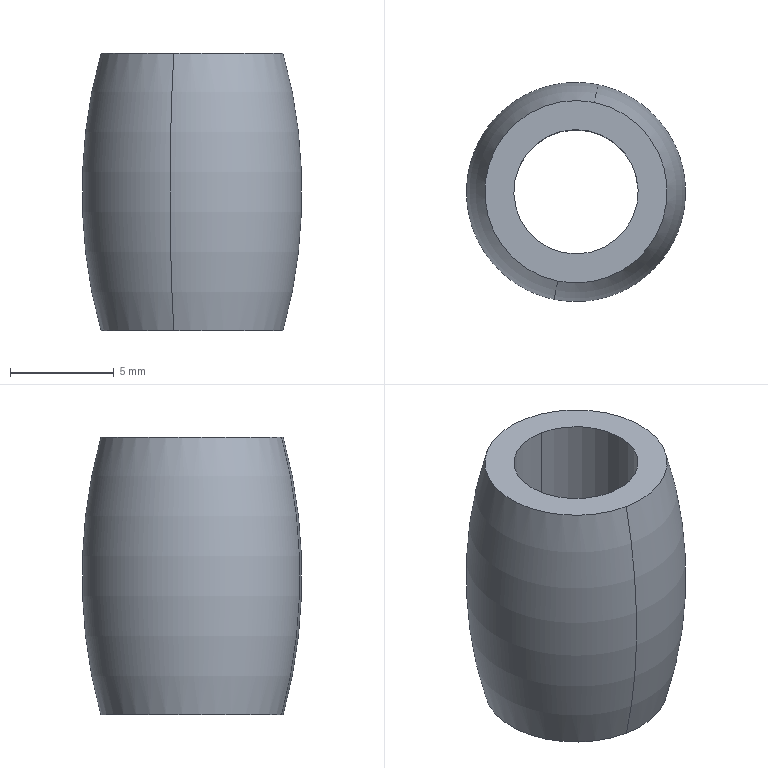Component | SolidWorks | Half-1_Roller-2 | 1 solid | 6 faces | volume 678 mm3 | cylinder 2 | plane 2 | torus 2 | commonest cylinder face diameters 6 x2 | material Rubber
build123d program:
from build123d import *

# Parameters (mm, degrees)
SKETCH2_R          = 3
CUT_EXTRUDE3_DEPTH = 30.203


with BuildPart() as part:
    # Sketch1 → Revolve1 (revolve)
    with BuildSketch(Plane.XY):
        with BuildLine():
            Line((-47.251, 20.1), (-33.851, 20.1))
            Line((-33.851, 20.1), (-33.851, 24.5))
            ThreePointArc((-33.851, 24.5), (-40.551, 25.4), (-47.251, 24.5))
            Line((-47.251, 24.5), (-47.251, 20.1))
        make_face()
    revolve(axis=Axis((-1.751, 20.1, 0), (-1, 0, 0)))

    # Sketch2 → Cut-Extrude3 (cut, through all)
    with BuildSketch(Plane(origin=(-33.851, 0, 0), x_dir=(0, 0, -1), z_dir=(1, 0, 0))):
        with Locations(Location((0, 20.1, 0), (0, 0, 90))):
            Circle(SKETCH2_R)
    extrude(amount=-CUT_EXTRUDE3_DEPTH, mode=Mode.SUBTRACT)


solid = part.part

# Placed as in the assembly
solid = solid.moved(Location((-19.269, -22.2, -3.551), (0, 90, 0)))
STEP:
#1=CARTESIAN_POINT('',(-0.7822,-0.1984,1.193));
#2=VERTEX_POINT('',#1);
#3=CARTESIAN_POINT('',(-0.735,0.03304,1.193));
#4=VERTEX_POINT('',#3);
#5=CARTESIAN_POINT('',(-0.7586,-0.08269,1.193));
#6=DIRECTION('',(-0.,-0.,1.));
#7=DIRECTION('',(0.1999,0.9798,0.));
#8=AXIS2_PLACEMENT_3D('',#5,#6,#7);
#9=CIRCLE('',#8,0.1181);
#10=EDGE_CURVE('',#2,#4,#9,.T.);
#11=ORIENTED_EDGE('',*,*,#10,.F.);
#12=CARTESIAN_POINT('',(-0.7822,-0.1984,1.72));
#13=VERTEX_POINT('',#12);
#14=CARTESIAN_POINT('',(-0.7822,-0.1984,1.193));
#15=DIRECTION('',(-0.,-0.,1.));
#16=VECTOR('',#15,39.37);
#17=LINE('',#14,#16);
#18=EDGE_CURVE('',#2,#13,#17,.T.);
#19=ORIENTED_EDGE('',*,*,#18,.T.);
#20=CARTESIAN_POINT('',(-0.735,0.03304,1.72));
#21=VERTEX_POINT('',#20);
#22=CARTESIAN_POINT('',(-0.7586,-0.08269,1.72));
#23=DIRECTION('',(-0.,-0.,1.));
#24=DIRECTION('',(0.1999,0.9798,0.));
#25=AXIS2_PLACEMENT_3D('',#22,#23,#24);
#26=CIRCLE('',#25,0.1181);
#27=EDGE_CURVE('',#13,#21,#26,.T.);
#28=ORIENTED_EDGE('',*,*,#27,.T.);
#29=CARTESIAN_POINT('',(-0.735,0.03304,1.193));
#30=DIRECTION('',(-0.,-0.,1.));
#31=VECTOR('',#30,39.37);
#32=LINE('',#29,#31);
#33=EDGE_CURVE('',#4,#21,#32,.T.);
#34=ORIENTED_EDGE('',*,*,#33,.F.);
#35=EDGE_LOOP('',(#11,#19,#28,#34));
#36=FACE_OUTER_BOUND('',#35,.T.);
#37=CARTESIAN_POINT('',(-0.7586,-0.08269,1.193));
#38=DIRECTION('',(-0.,-0.,1.));
#39=DIRECTION('',(0.1999,0.9798,0.));
#40=AXIS2_PLACEMENT_3D('',#37,#38,#39);
#41=CYLINDRICAL_SURFACE('',#40,0.1181);
#42=ADVANCED_FACE('',(#36),#41,.F.);
#43=CARTESIAN_POINT('',(-0.724,0.08706,1.193));
#44=VERTEX_POINT('',#43);
#45=CARTESIAN_POINT('',(-0.7933,-0.2524,1.193));
#46=VERTEX_POINT('',#45);
#47=CARTESIAN_POINT('',(-0.7586,-0.08269,1.193));
#48=DIRECTION('',(-0.,-0.,1.));
#49=DIRECTION('',(0.1999,0.9798,0.));
#50=AXIS2_PLACEMENT_3D('',#47,#48,#49);
#51=CIRCLE('',#50,0.1732);
#52=EDGE_CURVE('',#44,#46,#51,.T.);
#53=ORIENTED_EDGE('',*,*,#52,.T.);
#54=CARTESIAN_POINT('',(-0.7933,-0.2524,1.72));
#55=VERTEX_POINT('',#54);
#56=CARTESIAN_POINT('',(-0.6004,0.6927,1.457));
#57=DIRECTION('',(-0.9798,0.1999,-0.));
#58=DIRECTION('',(-0.1999,-0.9798,0.));
#59=AXIS2_PLACEMENT_3D('',#56,#57,#58);
#60=CIRCLE('',#59,1.);
#61=EDGE_CURVE('',#46,#55,#60,.T.);
#62=ORIENTED_EDGE('',*,*,#61,.T.);
#63=CARTESIAN_POINT('',(-0.724,0.08706,1.72));
#64=VERTEX_POINT('',#63);
#65=CARTESIAN_POINT('',(-0.7586,-0.08269,1.72));
#66=DIRECTION('',(-0.,-0.,1.));
#67=DIRECTION('',(0.1999,0.9798,0.));
#68=AXIS2_PLACEMENT_3D('',#65,#66,#67);
#69=CIRCLE('',#68,0.1732);
#70=EDGE_CURVE('',#64,#55,#69,.T.);
#71=ORIENTED_EDGE('',*,*,#70,.F.);
#72=CARTESIAN_POINT('',(-0.9168,-0.8581,1.457));
#73=DIRECTION('',(0.9798,-0.1999,0.));
#74=DIRECTION('',(0.1999,0.9798,0.));
#75=AXIS2_PLACEMENT_3D('',#72,#73,#74);
#76=CIRCLE('',#75,1.);
#77=EDGE_CURVE('',#44,#64,#76,.T.);
#78=ORIENTED_EDGE('',*,*,#77,.F.);
#79=EDGE_LOOP('',(#53,#62,#71,#78));
#80=FACE_OUTER_BOUND('',#79,.T.);
#81=CARTESIAN_POINT('',(-0.7586,-0.08269,1.457));
#82=DIRECTION('',(-0.,-0.,1.));
#83=DIRECTION('',(0.1999,0.9798,0.));
#84=AXIS2_PLACEMENT_3D('',#81,#82,#83);
#85=TOROIDAL_SURFACE('',#84,-0.7913,1.);
#86=ADVANCED_FACE('',(#80),#85,.T.);
#87=CARTESIAN_POINT('',(-0.7586,-0.08269,1.72));
#88=DIRECTION('',(-0.,-0.,1.));
#89=DIRECTION('',(0.1999,0.9798,0.));
#90=AXIS2_PLACEMENT_3D('',#87,#88,#89);
#91=CIRCLE('',#90,0.1181);
#92=EDGE_CURVE('',#21,#13,#91,.T.);
#93=ORIENTED_EDGE('',*,*,#92,.F.);
#94=ORIENTED_EDGE('',*,*,#27,.F.);
#95=EDGE_LOOP('',(#93,#94));
#96=FACE_BOUND('',#95,.T.);
#97=ORIENTED_EDGE('',*,*,#70,.T.);
#98=CARTESIAN_POINT('',(-0.7586,-0.08269,1.72));
#99=DIRECTION('',(-0.,-0.,1.));
#100=DIRECTION('',(0.1999,0.9798,0.));
#101=AXIS2_PLACEMENT_3D('',#98,#99,#100);
#102=CIRCLE('',#101,0.1732);
#103=EDGE_CURVE('',#55,#64,#102,.T.);
#104=ORIENTED_EDGE('',*,*,#103,.T.);
#105=EDGE_LOOP('',(#97,#104));
#106=FACE_OUTER_BOUND('',#105,.T.);
#107=CARTESIAN_POINT('',(-0.9168,-0.8581,1.72));
#108=DIRECTION('',(-0.,-0.,1.));
#109=DIRECTION('',(0.1999,0.9798,0.));
#110=AXIS2_PLACEMENT_3D('',#107,#108,#109);
#111=PLANE('',#110);
#112=ADVANCED_FACE('',(#96,#106),#111,.T.);
#113=ORIENTED_EDGE('',*,*,#61,.F.);
#114=CARTESIAN_POINT('',(-0.7586,-0.08269,1.193));
#115=DIRECTION('',(-0.,-0.,1.));
#116=DIRECTION('',(0.1999,0.9798,0.));
#117=AXIS2_PLACEMENT_3D('',#114,#115,#116);
#118=CIRCLE('',#117,0.1732);
#119=EDGE_CURVE('',#46,#44,#118,.T.);
#120=ORIENTED_EDGE('',*,*,#119,.T.);
#121=ORIENTED_EDGE('',*,*,#77,.T.);
#122=ORIENTED_EDGE('',*,*,#103,.F.);
#123=EDGE_LOOP('',(#113,#120,#121,#122));
#124=FACE_OUTER_BOUND('',#123,.T.);
#125=CARTESIAN_POINT('',(-0.7586,-0.08269,1.457));
#126=DIRECTION('',(-0.,-0.,1.));
#127=DIRECTION('',(0.1999,0.9798,0.));
#128=AXIS2_PLACEMENT_3D('',#125,#126,#127);
#129=TOROIDAL_SURFACE('',#128,-0.7913,1.);
#130=ADVANCED_FACE('',(#124),#129,.T.);
#131=CARTESIAN_POINT('',(-0.7586,-0.08269,1.193));
#132=DIRECTION('',(-0.,-0.,1.));
#133=DIRECTION('',(0.1999,0.9798,0.));
#134=AXIS2_PLACEMENT_3D('',#131,#132,#133);
#135=CIRCLE('',#134,0.1181);
#136=EDGE_CURVE('',#4,#2,#135,.T.);
#137=ORIENTED_EDGE('',*,*,#136,.T.);
#138=ORIENTED_EDGE('',*,*,#10,.T.);
#139=EDGE_LOOP('',(#137,#138));
#140=FACE_BOUND('',#139,.T.);
#141=ORIENTED_EDGE('',*,*,#52,.F.);
#142=ORIENTED_EDGE('',*,*,#119,.F.);
#143=EDGE_LOOP('',(#141,#142));
#144=FACE_OUTER_BOUND('',#143,.T.);
#145=CARTESIAN_POINT('',(-0.9168,-0.8581,1.193));
#146=DIRECTION('',(-0.,-0.,1.));
#147=DIRECTION('',(0.1999,0.9798,0.));
#148=AXIS2_PLACEMENT_3D('',#145,#146,#147);
#149=PLANE('',#148);
#150=ADVANCED_FACE('',(#140,#144),#149,.F.);
#151=ORIENTED_EDGE('',*,*,#18,.F.);
#152=ORIENTED_EDGE('',*,*,#136,.F.);
#153=ORIENTED_EDGE('',*,*,#33,.T.);
#154=ORIENTED_EDGE('',*,*,#92,.T.);
#155=EDGE_LOOP('',(#151,#152,#153,#154));
#156=FACE_OUTER_BOUND('',#155,.T.);
#157=CARTESIAN_POINT('',(-0.7586,-0.08269,1.193));
#158=DIRECTION('',(-0.,-0.,1.));
#159=DIRECTION('',(0.1999,0.9798,0.));
#160=AXIS2_PLACEMENT_3D('',#157,#158,#159);
#161=CYLINDRICAL_SURFACE('',#160,0.1181);
#162=ADVANCED_FACE('',(#156),#161,.F.);
#163=CLOSED_SHELL('',(#42,#86,#112,#130,#150,#162));
#164=MANIFOLD_SOLID_BREP('',#163);
#165=CARTESIAN_POINT('',(0.,0.,0.));
#166=DIRECTION('',(0.,0.,1.));
#167=DIRECTION('',(1.,0.,0.));
#168=AXIS2_PLACEMENT_3D('',#165,#166,#167);
#169=(LENGTH_UNIT()NAMED_UNIT(*)SI_UNIT($,.METRE.));
#170=LENGTH_MEASURE_WITH_UNIT(LENGTH_MEASURE(0.0254),#169);
#171=DIMENSIONAL_EXPONENTS(1.,0.,0.,0.,0.,0.,0.);
#172=(CONVERSION_BASED_UNIT('',#170)LENGTH_UNIT()NAMED_UNIT(#171));
#173=UNCERTAINTY_MEASURE_WITH_UNIT(LENGTH_MEASURE(0.00001),#172,'','');
#174=(NAMED_UNIT(*)PLANE_ANGLE_UNIT()SI_UNIT($,.RADIAN.));
#175=(NAMED_UNIT(*)SI_UNIT($,.STERADIAN.)SOLID_ANGLE_UNIT());
#176=(GEOMETRIC_REPRESENTATION_CONTEXT(3)GLOBAL_UNCERTAINTY_ASSIGNED_CONTEXT((#173))GLOBAL_UNIT_ASSIGNED_CONTEXT((#172,#174,#175))REPRESENTATION_CONTEXT('',''));
#177=ADVANCED_BREP_SHAPE_REPRESENTATION('',(#164,#168),#176);
#178=COLOUR_RGB('',0.7922,0.8196,0.9333);
#179=FILL_AREA_STYLE_COLOUR('',#178);
#180=FILL_AREA_STYLE('',(#179));
#181=SURFACE_STYLE_FILL_AREA(#180);
#182=SURFACE_SIDE_STYLE('',(#181));
#183=SURFACE_STYLE_USAGE(.BOTH.,#182);
#184=PRESENTATION_STYLE_ASSIGNMENT((#183));
#185=STYLED_ITEM('',(#184),#164);
#186=(LENGTH_UNIT()NAMED_UNIT(*)SI_UNIT($,.METRE.));
#187=LENGTH_MEASURE_WITH_UNIT(LENGTH_MEASURE(0.0254),#186);
#188=DIMENSIONAL_EXPONENTS(1.,0.,0.,0.,0.,0.,0.);
#189=(CONVERSION_BASED_UNIT('',#187)LENGTH_UNIT()NAMED_UNIT(#188));
#190=UNCERTAINTY_MEASURE_WITH_UNIT(LENGTH_MEASURE(0.00001),#189,'','');
#191=(NAMED_UNIT(*)PLANE_ANGLE_UNIT()SI_UNIT($,.RADIAN.));
#192=(NAMED_UNIT(*)SI_UNIT($,.STERADIAN.)SOLID_ANGLE_UNIT());
#193=(GEOMETRIC_REPRESENTATION_CONTEXT(3)GLOBAL_UNCERTAINTY_ASSIGNED_CONTEXT((#190))GLOBAL_UNIT_ASSIGNED_CONTEXT((#189,#191,#192))REPRESENTATION_CONTEXT('',''));
#194=MECHANICAL_DESIGN_GEOMETRIC_PRESENTATION_REPRESENTATION('',(#185),#193);
#195=PRESENTATION_LAYER_ASSIGNMENT('','',(#185));